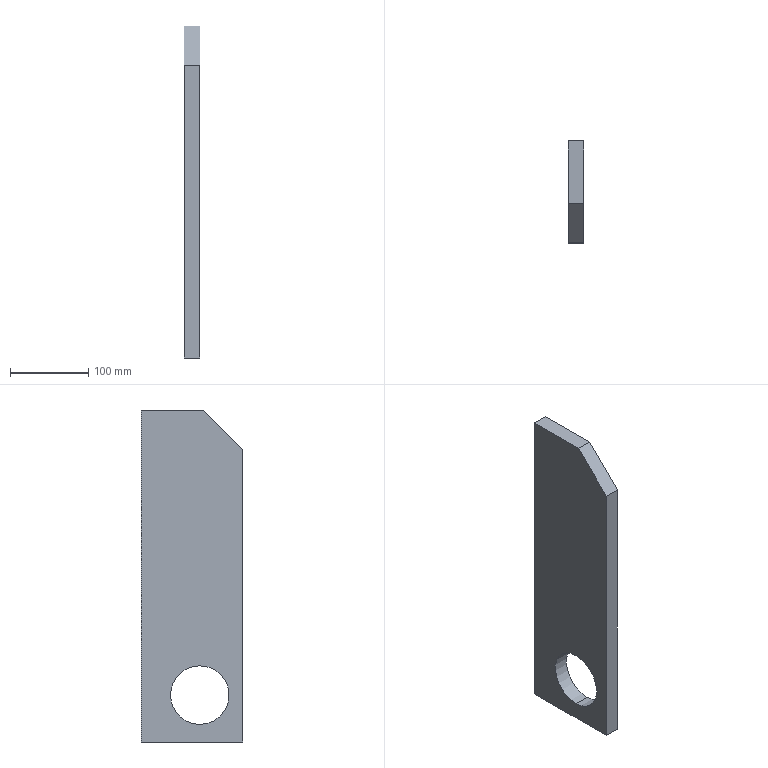Component | SolidWorks | JF21-80.1-1-3(_)-1-SOLID62-1 | 1 solid | 17 faces | box 20 x 130 x 425 mm | volume 988766 mm3 | plane 7 | cylinder 6 | cone 4 | commonest cylinder face diameters 8.5 x4 75 x2
STEP:
#1=COLOUR_RGB('',0.7922,0.8196,0.9333);
#2=FILL_AREA_STYLE_COLOUR('',#1);
#3=FILL_AREA_STYLE('',(#2));
#4=SURFACE_STYLE_FILL_AREA(#3);
#5=SURFACE_SIDE_STYLE('',(#4));
#6=SURFACE_STYLE_USAGE(.BOTH.,#5);
#7=PRESENTATION_STYLE_ASSIGNMENT((#6));
#8=CARTESIAN_POINT('',(-15.748,13.583,-6.201));
#9=VERTEX_POINT('',#8);
#10=CARTESIAN_POINT('',(-15.748,13.583,-3.248));
#11=VERTEX_POINT('',#10);
#12=CARTESIAN_POINT('',(-15.748,13.583,-4.724));
#13=DIRECTION('',(-1.,0.,0.));
#14=DIRECTION('',(0.,0.,1.));
#15=AXIS2_PLACEMENT_3D('',#12,#13,#14);
#16=CIRCLE('',#15,1.476);
#17=EDGE_CURVE('',#9,#11,#16,.T.);
#18=ORIENTED_EDGE('',*,*,#17,.T.);
#19=CARTESIAN_POINT('',(-14.961,13.583,-3.248));
#20=VERTEX_POINT('',#19);
#21=CARTESIAN_POINT('',(-21.654,13.583,-3.248));
#22=DIRECTION('',(-1.,0.,0.));
#23=VECTOR('',#22,39.37);
#24=LINE('',#21,#23);
#25=EDGE_CURVE('',#20,#11,#24,.T.);
#26=ORIENTED_EDGE('',*,*,#25,.F.);
#27=CARTESIAN_POINT('',(-14.961,13.583,-6.201));
#28=VERTEX_POINT('',#27);
#29=CARTESIAN_POINT('',(-14.961,13.583,-4.724));
#30=DIRECTION('',(1.,0.,0.));
#31=DIRECTION('',(0.,0.,-1.));
#32=AXIS2_PLACEMENT_3D('',#29,#30,#31);
#33=CIRCLE('',#32,1.476);
#34=EDGE_CURVE('',#20,#28,#33,.T.);
#35=ORIENTED_EDGE('',*,*,#34,.T.);
#36=CARTESIAN_POINT('',(-21.654,13.583,-6.201));
#37=DIRECTION('',(-1.,0.,0.));
#38=VECTOR('',#37,39.37);
#39=LINE('',#36,#38);
#40=EDGE_CURVE('',#28,#9,#39,.T.);
#41=ORIENTED_EDGE('',*,*,#40,.T.);
#42=EDGE_LOOP('',(#18,#26,#35,#41));
#43=FACE_OUTER_BOUND('',#42,.T.);
#44=CARTESIAN_POINT('',(-21.654,13.583,-4.724));
#45=DIRECTION('',(1.,0.,0.));
#46=DIRECTION('',(0.,0.,1.));
#47=AXIS2_PLACEMENT_3D('',#44,#45,#46);
#48=CYLINDRICAL_SURFACE('',#47,1.476);
#49=ADVANCED_FACE('',(#43),#48,.F.);
#50=CARTESIAN_POINT('',(-15.453,15.571,1.703));
#51=VERTEX_POINT('',#50);
#52=CARTESIAN_POINT('',(-15.453,15.571,2.037));
#53=VERTEX_POINT('',#52);
#54=CARTESIAN_POINT('',(-15.453,15.571,1.87));
#55=DIRECTION('',(0.,1.,0.));
#56=DIRECTION('',(0.,0.,1.));
#57=AXIS2_PLACEMENT_3D('',#54,#55,#56);
#58=CIRCLE('',#57,0.1673);
#59=EDGE_CURVE('',#51,#53,#58,.T.);
#60=ORIENTED_EDGE('',*,*,#59,.F.);
#61=CARTESIAN_POINT('',(-15.453,16.535,1.703));
#62=VERTEX_POINT('',#61);
#63=CARTESIAN_POINT('',(-15.453,16.535,1.703));
#64=DIRECTION('',(0.,1.,0.));
#65=VECTOR('',#64,39.37);
#66=LINE('',#63,#65);
#67=EDGE_CURVE('',#51,#62,#66,.T.);
#68=ORIENTED_EDGE('',*,*,#67,.T.);
#69=CARTESIAN_POINT('',(-15.453,16.535,2.037));
#70=VERTEX_POINT('',#69);
#71=CARTESIAN_POINT('',(-15.453,16.535,1.87));
#72=DIRECTION('',(0.,1.,0.));
#73=DIRECTION('',(0.,0.,1.));
#74=AXIS2_PLACEMENT_3D('',#71,#72,#73);
#75=CIRCLE('',#74,0.1673);
#76=EDGE_CURVE('',#62,#70,#75,.T.);
#77=ORIENTED_EDGE('',*,*,#76,.T.);
#78=CARTESIAN_POINT('',(-15.453,16.535,2.037));
#79=DIRECTION('',(0.,1.,0.));
#80=VECTOR('',#79,39.37);
#81=LINE('',#78,#80);
#82=EDGE_CURVE('',#53,#70,#81,.T.);
#83=ORIENTED_EDGE('',*,*,#82,.F.);
#84=EDGE_LOOP('',(#60,#68,#77,#83));
#85=FACE_OUTER_BOUND('',#84,.T.);
#86=CARTESIAN_POINT('',(-15.453,16.535,1.87));
#87=DIRECTION('',(0.,1.,0.));
#88=DIRECTION('',(0.,0.,-1.));
#89=AXIS2_PLACEMENT_3D('',#86,#87,#88);
#90=CYLINDRICAL_SURFACE('',#89,0.1673);
#91=ADVANCED_FACE('',(#85),#90,.F.);
#92=CARTESIAN_POINT('',(-15.453,15.47,1.87));
#93=VERTEX_POINT('',#92);
#94=CARTESIAN_POINT('',(-15.453,15.571,2.037));
#95=DIRECTION('',(0.,0.515,0.8572));
#96=VECTOR('',#95,39.37);
#97=LINE('',#94,#96);
#98=EDGE_CURVE('',#93,#53,#97,.T.);
#99=ORIENTED_EDGE('',*,*,#98,.F.);
#100=CARTESIAN_POINT('',(-15.453,15.571,1.703));
#101=DIRECTION('',(0.,0.515,-0.8572));
#102=VECTOR('',#101,39.37);
#103=LINE('',#100,#102);
#104=EDGE_CURVE('',#93,#51,#103,.T.);
#105=ORIENTED_EDGE('',*,*,#104,.T.);
#106=ORIENTED_EDGE('',*,*,#59,.T.);
#107=EDGE_LOOP('',(#99,#105,#106));
#108=FACE_OUTER_BOUND('',#107,.T.);
#109=CARTESIAN_POINT('',(-15.453,15.571,1.87));
#110=DIRECTION('',(0.,1.,0.));
#111=DIRECTION('',(0.,0.,-1.));
#112=AXIS2_PLACEMENT_3D('',#109,#110,#111);
#113=CONICAL_SURFACE('',#112,0.1673,1.03);
#114=ADVANCED_FACE('',(#108),#113,.F.);
#115=CARTESIAN_POINT('',(-15.453,15.571,8.199));
#116=VERTEX_POINT('',#115);
#117=CARTESIAN_POINT('',(-15.453,15.571,8.533));
#118=VERTEX_POINT('',#117);
#119=CARTESIAN_POINT('',(-15.453,15.571,8.366));
#120=DIRECTION('',(0.,1.,0.));
#121=DIRECTION('',(0.,0.,1.));
#122=AXIS2_PLACEMENT_3D('',#119,#120,#121);
#123=CIRCLE('',#122,0.1673);
#124=EDGE_CURVE('',#116,#118,#123,.T.);
#125=ORIENTED_EDGE('',*,*,#124,.F.);
#126=CARTESIAN_POINT('',(-15.453,16.535,8.199));
#127=VERTEX_POINT('',#126);
#128=CARTESIAN_POINT('',(-15.453,16.535,8.199));
#129=DIRECTION('',(0.,1.,0.));
#130=VECTOR('',#129,39.37);
#131=LINE('',#128,#130);
#132=EDGE_CURVE('',#116,#127,#131,.T.);
#133=ORIENTED_EDGE('',*,*,#132,.T.);
#134=CARTESIAN_POINT('',(-15.453,16.535,8.533));
#135=VERTEX_POINT('',#134);
#136=CARTESIAN_POINT('',(-15.453,16.535,8.366));
#137=DIRECTION('',(0.,1.,0.));
#138=DIRECTION('',(0.,0.,1.));
#139=AXIS2_PLACEMENT_3D('',#136,#137,#138);
#140=CIRCLE('',#139,0.1673);
#141=EDGE_CURVE('',#127,#135,#140,.T.);
#142=ORIENTED_EDGE('',*,*,#141,.T.);
#143=CARTESIAN_POINT('',(-15.453,16.535,8.533));
#144=DIRECTION('',(0.,1.,0.));
#145=VECTOR('',#144,39.37);
#146=LINE('',#143,#145);
#147=EDGE_CURVE('',#118,#135,#146,.T.);
#148=ORIENTED_EDGE('',*,*,#147,.F.);
#149=EDGE_LOOP('',(#125,#133,#142,#148));
#150=FACE_OUTER_BOUND('',#149,.T.);
#151=CARTESIAN_POINT('',(-15.453,16.535,8.366));
#152=DIRECTION('',(0.,1.,0.));
#153=DIRECTION('',(0.,0.,-1.));
#154=AXIS2_PLACEMENT_3D('',#151,#152,#153);
#155=CYLINDRICAL_SURFACE('',#154,0.1673);
#156=ADVANCED_FACE('',(#150),#155,.F.);
#157=CARTESIAN_POINT('',(-15.453,15.47,8.366));
#158=VERTEX_POINT('',#157);
#159=CARTESIAN_POINT('',(-15.453,15.571,8.533));
#160=DIRECTION('',(0.,0.515,0.8572));
#161=VECTOR('',#160,39.37);
#162=LINE('',#159,#161);
#163=EDGE_CURVE('',#158,#118,#162,.T.);
#164=ORIENTED_EDGE('',*,*,#163,.F.);
#165=CARTESIAN_POINT('',(-15.453,15.571,8.199));
#166=DIRECTION('',(0.,0.515,-0.8572));
#167=VECTOR('',#166,39.37);
#168=LINE('',#165,#167);
#169=EDGE_CURVE('',#158,#116,#168,.T.);
#170=ORIENTED_EDGE('',*,*,#169,.T.);
#171=ORIENTED_EDGE('',*,*,#124,.T.);
#172=EDGE_LOOP('',(#164,#170,#171));
#173=FACE_OUTER_BOUND('',#172,.T.);
#174=CARTESIAN_POINT('',(-15.453,15.571,8.366));
#175=DIRECTION('',(0.,1.,0.));
#176=DIRECTION('',(0.,0.,-1.));
#177=AXIS2_PLACEMENT_3D('',#174,#175,#176);
#178=CONICAL_SURFACE('',#177,0.1673,1.03);
#179=ADVANCED_FACE('',(#173),#178,.F.);
#180=ORIENTED_EDGE('',*,*,#17,.F.);
#181=CARTESIAN_POINT('',(-15.748,13.583,-4.724));
#182=DIRECTION('',(-1.,0.,0.));
#183=DIRECTION('',(0.,0.,1.));
#184=AXIS2_PLACEMENT_3D('',#181,#182,#183);
#185=CIRCLE('',#184,1.476);
#186=EDGE_CURVE('',#11,#9,#185,.T.);
#187=ORIENTED_EDGE('',*,*,#186,.F.);
#188=EDGE_LOOP('',(#180,#187));
#189=FACE_BOUND('',#188,.T.);
#190=CARTESIAN_POINT('',(-15.748,11.417,-7.087));
#191=VERTEX_POINT('',#190);
#192=CARTESIAN_POINT('',(-15.748,11.417,7.677));
#193=VERTEX_POINT('',#192);
#194=CARTESIAN_POINT('',(-15.748,11.417,-7.087));
#195=DIRECTION('',(0.,0.,1.));
#196=VECTOR('',#195,39.37);
#197=LINE('',#194,#196);
#198=EDGE_CURVE('',#191,#193,#197,.T.);
#199=ORIENTED_EDGE('',*,*,#198,.T.);
#200=CARTESIAN_POINT('',(-15.748,13.386,9.646));
#201=VERTEX_POINT('',#200);
#202=CARTESIAN_POINT('',(-15.748,4.035,0.2953));
#203=DIRECTION('',(0.,0.7071,0.7071));
#204=VECTOR('',#203,39.37);
#205=LINE('',#202,#204);
#206=EDGE_CURVE('',#193,#201,#205,.T.);
#207=ORIENTED_EDGE('',*,*,#206,.T.);
#208=CARTESIAN_POINT('',(-15.748,16.535,9.646));
#209=VERTEX_POINT('',#208);
#210=CARTESIAN_POINT('',(-15.748,11.417,9.646));
#211=DIRECTION('',(0.,1.,0.));
#212=VECTOR('',#211,39.37);
#213=LINE('',#210,#212);
#214=EDGE_CURVE('',#201,#209,#213,.T.);
#215=ORIENTED_EDGE('',*,*,#214,.T.);
#216=CARTESIAN_POINT('',(-15.748,16.535,-7.087));
#217=VERTEX_POINT('',#216);
#218=CARTESIAN_POINT('',(-15.748,16.535,-7.087));
#219=DIRECTION('',(0.,0.,1.));
#220=VECTOR('',#219,39.37);
#221=LINE('',#218,#220);
#222=EDGE_CURVE('',#217,#209,#221,.T.);
#223=ORIENTED_EDGE('',*,*,#222,.F.);
#224=CARTESIAN_POINT('',(-15.748,11.417,-7.087));
#225=DIRECTION('',(0.,1.,0.));
#226=VECTOR('',#225,39.37);
#227=LINE('',#224,#226);
#228=EDGE_CURVE('',#191,#217,#227,.T.);
#229=ORIENTED_EDGE('',*,*,#228,.F.);
#230=EDGE_LOOP('',(#199,#207,#215,#223,#229));
#231=FACE_OUTER_BOUND('',#230,.T.);
#232=CARTESIAN_POINT('',(-15.748,11.417,-7.087));
#233=DIRECTION('',(-1.,0.,0.));
#234=DIRECTION('',(0.,0.,-1.));
#235=AXIS2_PLACEMENT_3D('',#232,#233,#234);
#236=PLANE('',#235);
#237=ADVANCED_FACE('',(#189,#231),#236,.T.);
#238=CARTESIAN_POINT('',(-14.961,16.535,-7.087));
#239=VERTEX_POINT('',#238);
#240=CARTESIAN_POINT('',(-15.748,16.535,-7.087));
#241=DIRECTION('',(-1.,0.,0.));
#242=VECTOR('',#241,39.37);
#243=LINE('',#240,#242);
#244=EDGE_CURVE('',#239,#217,#243,.T.);
#245=ORIENTED_EDGE('',*,*,#244,.F.);
#246=CARTESIAN_POINT('',(-14.961,11.417,-7.087));
#247=VERTEX_POINT('',#246);
#248=CARTESIAN_POINT('',(-14.961,11.417,-7.087));
#249=DIRECTION('',(0.,1.,0.));
#250=VECTOR('',#249,39.37);
#251=LINE('',#248,#250);
#252=EDGE_CURVE('',#247,#239,#251,.T.);
#253=ORIENTED_EDGE('',*,*,#252,.F.);
#254=CARTESIAN_POINT('',(-15.748,11.417,-7.087));
#255=DIRECTION('',(-1.,0.,0.));
#256=VECTOR('',#255,39.37);
#257=LINE('',#254,#256);
#258=EDGE_CURVE('',#247,#191,#257,.T.);
#259=ORIENTED_EDGE('',*,*,#258,.T.);
#260=ORIENTED_EDGE('',*,*,#228,.T.);
#261=EDGE_LOOP('',(#245,#253,#259,#260));
#262=FACE_OUTER_BOUND('',#261,.T.);
#263=CARTESIAN_POINT('',(-15.748,11.417,-7.087));
#264=DIRECTION('',(0.,0.,-1.));
#265=DIRECTION('',(1.,0.,0.));
#266=AXIS2_PLACEMENT_3D('',#263,#264,#265);
#267=PLANE('',#266);
#268=ADVANCED_FACE('',(#262),#267,.T.);
#269=CARTESIAN_POINT('',(-14.961,13.583,-4.724));
#270=DIRECTION('',(1.,0.,0.));
#271=DIRECTION('',(0.,0.,-1.));
#272=AXIS2_PLACEMENT_3D('',#269,#270,#271);
#273=CIRCLE('',#272,1.476);
#274=EDGE_CURVE('',#28,#20,#273,.T.);
#275=ORIENTED_EDGE('',*,*,#274,.F.);
#276=ORIENTED_EDGE('',*,*,#34,.F.);
#277=EDGE_LOOP('',(#275,#276));
#278=FACE_BOUND('',#277,.T.);
#279=CARTESIAN_POINT('',(-14.961,13.386,9.646));
#280=VERTEX_POINT('',#279);
#281=CARTESIAN_POINT('',(-14.961,16.535,9.646));
#282=VERTEX_POINT('',#281);
#283=CARTESIAN_POINT('',(-14.961,11.417,9.646));
#284=DIRECTION('',(0.,1.,0.));
#285=VECTOR('',#284,39.37);
#286=LINE('',#283,#285);
#287=EDGE_CURVE('',#280,#282,#286,.T.);
#288=ORIENTED_EDGE('',*,*,#287,.F.);
#289=CARTESIAN_POINT('',(-14.961,11.417,7.677));
#290=VERTEX_POINT('',#289);
#291=CARTESIAN_POINT('',(-14.961,4.035,0.2953));
#292=DIRECTION('',(0.,-0.7071,-0.7071));
#293=VECTOR('',#292,39.37);
#294=LINE('',#291,#293);
#295=EDGE_CURVE('',#280,#290,#294,.T.);
#296=ORIENTED_EDGE('',*,*,#295,.T.);
#297=CARTESIAN_POINT('',(-14.961,11.417,-7.087));
#298=DIRECTION('',(0.,0.,-1.));
#299=VECTOR('',#298,39.37);
#300=LINE('',#297,#299);
#301=EDGE_CURVE('',#290,#247,#300,.T.);
#302=ORIENTED_EDGE('',*,*,#301,.T.);
#303=ORIENTED_EDGE('',*,*,#252,.T.);
#304=CARTESIAN_POINT('',(-14.961,16.535,-7.087));
#305=DIRECTION('',(0.,0.,-1.));
#306=VECTOR('',#305,39.37);
#307=LINE('',#304,#306);
#308=EDGE_CURVE('',#282,#239,#307,.T.);
#309=ORIENTED_EDGE('',*,*,#308,.F.);
#310=EDGE_LOOP('',(#288,#296,#302,#303,#309));
#311=FACE_OUTER_BOUND('',#310,.T.);
#312=CARTESIAN_POINT('',(-14.961,11.417,-7.087));
#313=DIRECTION('',(1.,0.,0.));
#314=DIRECTION('',(0.,0.,1.));
#315=AXIS2_PLACEMENT_3D('',#312,#313,#314);
#316=PLANE('',#315);
#317=ADVANCED_FACE('',(#278,#311),#316,.T.);
#318=ORIENTED_EDGE('',*,*,#214,.F.);
#319=CARTESIAN_POINT('',(-14.961,13.386,9.646));
#320=DIRECTION('',(1.,0.,0.));
#321=VECTOR('',#320,39.37);
#322=LINE('',#319,#321);
#323=EDGE_CURVE('',#201,#280,#322,.T.);
#324=ORIENTED_EDGE('',*,*,#323,.T.);
#325=ORIENTED_EDGE('',*,*,#287,.T.);
#326=CARTESIAN_POINT('',(-15.748,16.535,9.646));
#327=DIRECTION('',(1.,0.,0.));
#328=VECTOR('',#327,39.37);
#329=LINE('',#326,#328);
#330=EDGE_CURVE('',#209,#282,#329,.T.);
#331=ORIENTED_EDGE('',*,*,#330,.F.);
#332=EDGE_LOOP('',(#318,#324,#325,#331));
#333=FACE_OUTER_BOUND('',#332,.T.);
#334=CARTESIAN_POINT('',(-15.748,11.417,9.646));
#335=DIRECTION('',(0.,0.,1.));
#336=DIRECTION('',(-1.,0.,0.));
#337=AXIS2_PLACEMENT_3D('',#334,#335,#336);
#338=PLANE('',#337);
#339=ADVANCED_FACE('',(#333),#338,.T.);
#340=ORIENTED_EDGE('',*,*,#301,.F.);
#341=CARTESIAN_POINT('',(-15.748,11.417,7.677));
#342=DIRECTION('',(-1.,0.,0.));
#343=VECTOR('',#342,39.37);
#344=LINE('',#341,#343);
#345=EDGE_CURVE('',#290,#193,#344,.T.);
#346=ORIENTED_EDGE('',*,*,#345,.T.);
#347=ORIENTED_EDGE('',*,*,#198,.F.);
#348=ORIENTED_EDGE('',*,*,#258,.F.);
#349=EDGE_LOOP('',(#340,#346,#347,#348));
#350=FACE_OUTER_BOUND('',#349,.T.);
#351=CARTESIAN_POINT('',(-15.748,11.417,9.646));
#352=DIRECTION('',(0.,1.,0.));
#353=DIRECTION('',(0.,0.,-1.));
#354=AXIS2_PLACEMENT_3D('',#351,#352,#353);
#355=PLANE('',#354);
#356=ADVANCED_FACE('',(#350),#355,.F.);
#357=CARTESIAN_POINT('',(-15.453,16.535,1.87));
#358=DIRECTION('',(0.,1.,0.));
#359=DIRECTION('',(0.,0.,1.));
#360=AXIS2_PLACEMENT_3D('',#357,#358,#359);
#361=CIRCLE('',#360,0.1673);
#362=EDGE_CURVE('',#70,#62,#361,.T.);
#363=ORIENTED_EDGE('',*,*,#362,.F.);
#364=ORIENTED_EDGE('',*,*,#76,.F.);
#365=EDGE_LOOP('',(#363,#364));
#366=FACE_BOUND('',#365,.T.);
#367=CARTESIAN_POINT('',(-15.453,16.535,8.366));
#368=DIRECTION('',(0.,1.,0.));
#369=DIRECTION('',(0.,0.,1.));
#370=AXIS2_PLACEMENT_3D('',#367,#368,#369);
#371=CIRCLE('',#370,0.1673);
#372=EDGE_CURVE('',#135,#127,#371,.T.);
#373=ORIENTED_EDGE('',*,*,#372,.F.);
#374=ORIENTED_EDGE('',*,*,#141,.F.);
#375=EDGE_LOOP('',(#373,#374));
#376=FACE_BOUND('',#375,.T.);
#377=ORIENTED_EDGE('',*,*,#222,.T.);
#378=ORIENTED_EDGE('',*,*,#330,.T.);
#379=ORIENTED_EDGE('',*,*,#308,.T.);
#380=ORIENTED_EDGE('',*,*,#244,.T.);
#381=EDGE_LOOP('',(#377,#378,#379,#380));
#382=FACE_OUTER_BOUND('',#381,.T.);
#383=CARTESIAN_POINT('',(-15.748,16.535,9.646));
#384=DIRECTION('',(0.,1.,0.));
#385=DIRECTION('',(0.,0.,-1.));
#386=AXIS2_PLACEMENT_3D('',#383,#384,#385);
#387=PLANE('',#386);
#388=ADVANCED_FACE('',(#366,#376,#382),#387,.T.);
#389=ORIENTED_EDGE('',*,*,#206,.F.);
#390=ORIENTED_EDGE('',*,*,#345,.F.);
#391=ORIENTED_EDGE('',*,*,#295,.F.);
#392=ORIENTED_EDGE('',*,*,#323,.F.);
#393=EDGE_LOOP('',(#389,#390,#391,#392));
#394=FACE_OUTER_BOUND('',#393,.T.);
#395=CARTESIAN_POINT('',(-15.748,13.386,9.646));
#396=DIRECTION('',(0.,-0.7071,0.7071));
#397=DIRECTION('',(0.,0.7071,0.7071));
#398=AXIS2_PLACEMENT_3D('',#395,#396,#397);
#399=PLANE('',#398);
#400=ADVANCED_FACE('',(#394),#399,.T.);
#401=ORIENTED_EDGE('',*,*,#169,.F.);
#402=ORIENTED_EDGE('',*,*,#163,.T.);
#403=CARTESIAN_POINT('',(-15.453,15.571,8.366));
#404=DIRECTION('',(0.,1.,0.));
#405=DIRECTION('',(0.,0.,1.));
#406=AXIS2_PLACEMENT_3D('',#403,#404,#405);
#407=CIRCLE('',#406,0.1673);
#408=EDGE_CURVE('',#118,#116,#407,.T.);
#409=ORIENTED_EDGE('',*,*,#408,.T.);
#410=EDGE_LOOP('',(#401,#402,#409));
#411=FACE_OUTER_BOUND('',#410,.T.);
#412=CARTESIAN_POINT('',(-15.453,15.571,8.366));
#413=DIRECTION('',(0.,1.,0.));
#414=DIRECTION('',(0.,0.,-1.));
#415=AXIS2_PLACEMENT_3D('',#412,#413,#414);
#416=CONICAL_SURFACE('',#415,0.1673,1.03);
#417=ADVANCED_FACE('',(#411),#416,.F.);
#418=ORIENTED_EDGE('',*,*,#132,.F.);
#419=ORIENTED_EDGE('',*,*,#408,.F.);
#420=ORIENTED_EDGE('',*,*,#147,.T.);
#421=ORIENTED_EDGE('',*,*,#372,.T.);
#422=EDGE_LOOP('',(#418,#419,#420,#421));
#423=FACE_OUTER_BOUND('',#422,.T.);
#424=CARTESIAN_POINT('',(-15.453,16.535,8.366));
#425=DIRECTION('',(0.,1.,0.));
#426=DIRECTION('',(0.,0.,-1.));
#427=AXIS2_PLACEMENT_3D('',#424,#425,#426);
#428=CYLINDRICAL_SURFACE('',#427,0.1673);
#429=ADVANCED_FACE('',(#423),#428,.F.);
#430=ORIENTED_EDGE('',*,*,#104,.F.);
#431=ORIENTED_EDGE('',*,*,#98,.T.);
#432=CARTESIAN_POINT('',(-15.453,15.571,1.87));
#433=DIRECTION('',(0.,1.,0.));
#434=DIRECTION('',(0.,0.,1.));
#435=AXIS2_PLACEMENT_3D('',#432,#433,#434);
#436=CIRCLE('',#435,0.1673);
#437=EDGE_CURVE('',#53,#51,#436,.T.);
#438=ORIENTED_EDGE('',*,*,#437,.T.);
#439=EDGE_LOOP('',(#430,#431,#438));
#440=FACE_OUTER_BOUND('',#439,.T.);
#441=CARTESIAN_POINT('',(-15.453,15.571,1.87));
#442=DIRECTION('',(0.,1.,0.));
#443=DIRECTION('',(0.,0.,-1.));
#444=AXIS2_PLACEMENT_3D('',#441,#442,#443);
#445=CONICAL_SURFACE('',#444,0.1673,1.03);
#446=ADVANCED_FACE('',(#440),#445,.F.);
#447=ORIENTED_EDGE('',*,*,#67,.F.);
#448=ORIENTED_EDGE('',*,*,#437,.F.);
#449=ORIENTED_EDGE('',*,*,#82,.T.);
#450=ORIENTED_EDGE('',*,*,#362,.T.);
#451=EDGE_LOOP('',(#447,#448,#449,#450));
#452=FACE_OUTER_BOUND('',#451,.T.);
#453=CARTESIAN_POINT('',(-15.453,16.535,1.87));
#454=DIRECTION('',(0.,1.,0.));
#455=DIRECTION('',(0.,0.,-1.));
#456=AXIS2_PLACEMENT_3D('',#453,#454,#455);
#457=CYLINDRICAL_SURFACE('',#456,0.1673);
#458=ADVANCED_FACE('',(#452),#457,.F.);
#459=ORIENTED_EDGE('',*,*,#25,.T.);
#460=ORIENTED_EDGE('',*,*,#186,.T.);
#461=ORIENTED_EDGE('',*,*,#40,.F.);
#462=ORIENTED_EDGE('',*,*,#274,.T.);
#463=EDGE_LOOP('',(#459,#460,#461,#462));
#464=FACE_OUTER_BOUND('',#463,.T.);
#465=CARTESIAN_POINT('',(-21.654,13.583,-4.724));
#466=DIRECTION('',(1.,0.,0.));
#467=DIRECTION('',(0.,0.,1.));
#468=AXIS2_PLACEMENT_3D('',#465,#466,#467);
#469=CYLINDRICAL_SURFACE('',#468,1.476);
#470=ADVANCED_FACE('',(#464),#469,.F.);
#471=CLOSED_SHELL('',(#49,#91,#114,#156,#179,#237,#268,#317,#339,#356,#388,#400,#417,#429,#446,#458,#470));
#472=MANIFOLD_SOLID_BREP('',#471);
#473=STYLED_ITEM('',(#7),#472);
#474=(LENGTH_UNIT()NAMED_UNIT(*)SI_UNIT($,.METRE.));
#475=LENGTH_MEASURE_WITH_UNIT(LENGTH_MEASURE(0.0254),#474);
#476=DIMENSIONAL_EXPONENTS(1.,0.,0.,0.,0.,0.,0.);
#477=(CONVERSION_BASED_UNIT('',#475)LENGTH_UNIT()NAMED_UNIT(#476));
#478=UNCERTAINTY_MEASURE_WITH_UNIT(LENGTH_MEASURE(0.00001),#477,'','');
#479=(NAMED_UNIT(*)PLANE_ANGLE_UNIT()SI_UNIT($,.RADIAN.));
#480=(NAMED_UNIT(*)SI_UNIT($,.STERADIAN.)SOLID_ANGLE_UNIT());
#481=(GEOMETRIC_REPRESENTATION_CONTEXT(3)GLOBAL_UNCERTAINTY_ASSIGNED_CONTEXT((#478))GLOBAL_UNIT_ASSIGNED_CONTEXT((#477,#479,#480))REPRESENTATION_CONTEXT('',''));
#482=MECHANICAL_DESIGN_GEOMETRIC_PRESENTATION_REPRESENTATION('',(#473),#481);
#483=CARTESIAN_POINT('',(0.,0.,0.));
#484=DIRECTION('',(0.,0.,1.));
#485=DIRECTION('',(1.,0.,0.));
#486=AXIS2_PLACEMENT_3D('',#483,#484,#485);
#487=(LENGTH_UNIT()NAMED_UNIT(*)SI_UNIT($,.METRE.));
#488=LENGTH_MEASURE_WITH_UNIT(LENGTH_MEASURE(0.0254),#487);
#489=DIMENSIONAL_EXPONENTS(1.,0.,0.,0.,0.,0.,0.);
#490=(CONVERSION_BASED_UNIT('',#488)LENGTH_UNIT()NAMED_UNIT(#489));
#491=UNCERTAINTY_MEASURE_WITH_UNIT(LENGTH_MEASURE(0.00001),#490,'','');
#492=(NAMED_UNIT(*)PLANE_ANGLE_UNIT()SI_UNIT($,.RADIAN.));
#493=(NAMED_UNIT(*)SI_UNIT($,.STERADIAN.)SOLID_ANGLE_UNIT());
#494=(GEOMETRIC_REPRESENTATION_CONTEXT(3)GLOBAL_UNCERTAINTY_ASSIGNED_CONTEXT((#491))GLOBAL_UNIT_ASSIGNED_CONTEXT((#490,#492,#493))REPRESENTATION_CONTEXT('',''));
#495=ADVANCED_BREP_SHAPE_REPRESENTATION('',(#472,#486),#494);
#496=PRESENTATION_LAYER_ASSIGNMENT('','',(#473));